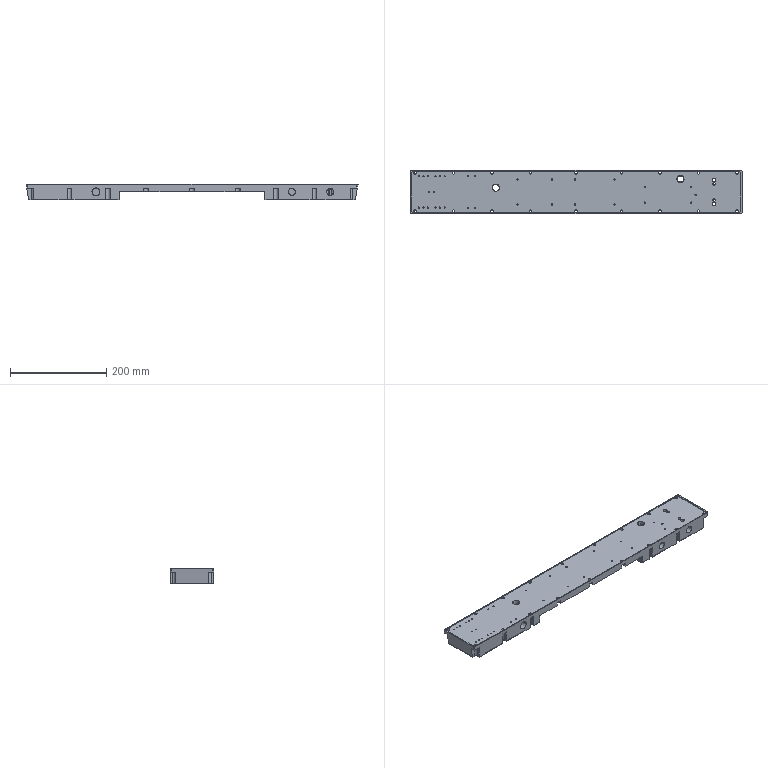CAM job | Mastercam | mm | 18 operations | part box 691.4 x 90 x 32.6
1. Facing | 24 - 100 平铣刀
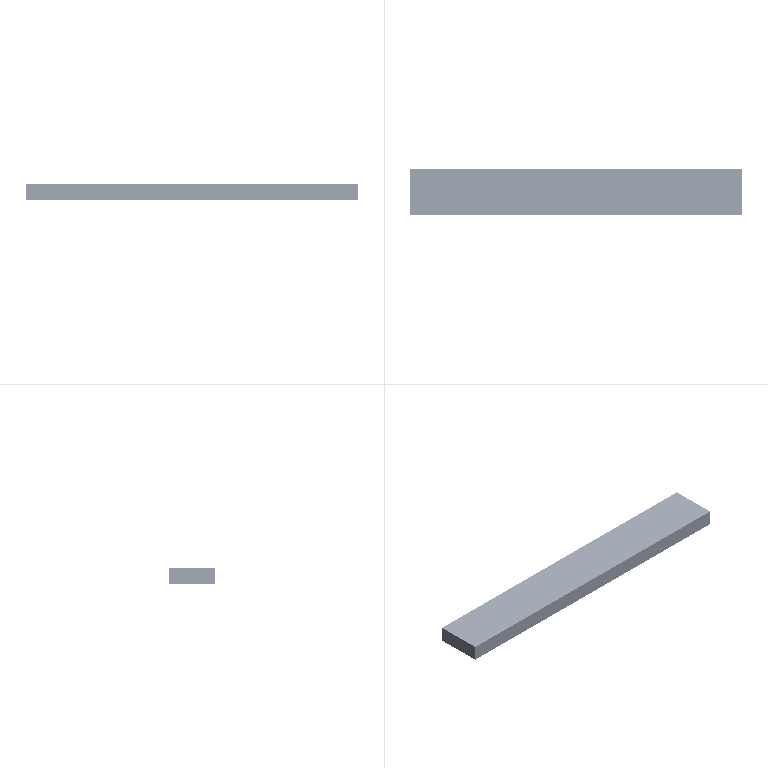2. 2D High Speed (2D Dynamic Mill) | 13 - 16 平铣刀
3. 2D High Speed (2D Area Mill) | 13 - 16 平铣刀
4. Contour (Remachining) | 8 - 8 平铣刀
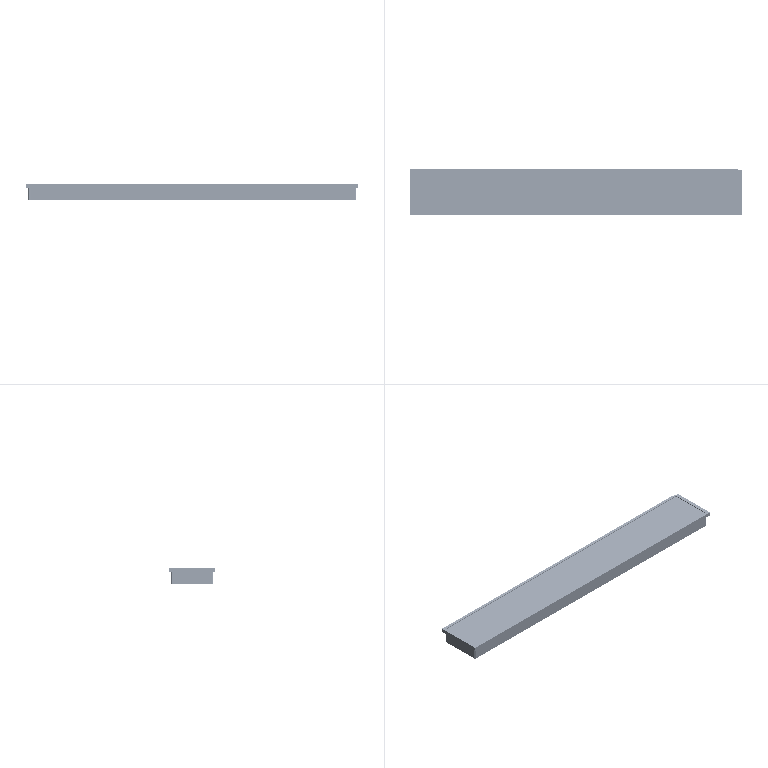5. 2D High Speed (2D Area Mill) | 8 - 8 平铣刀
6. Contour (2D) | 8 - 8 平铣刀
7. Contour (2D) | 16 - 16 平铣刀
8. Drill/Counterbore | 5 - 4 倒角刀
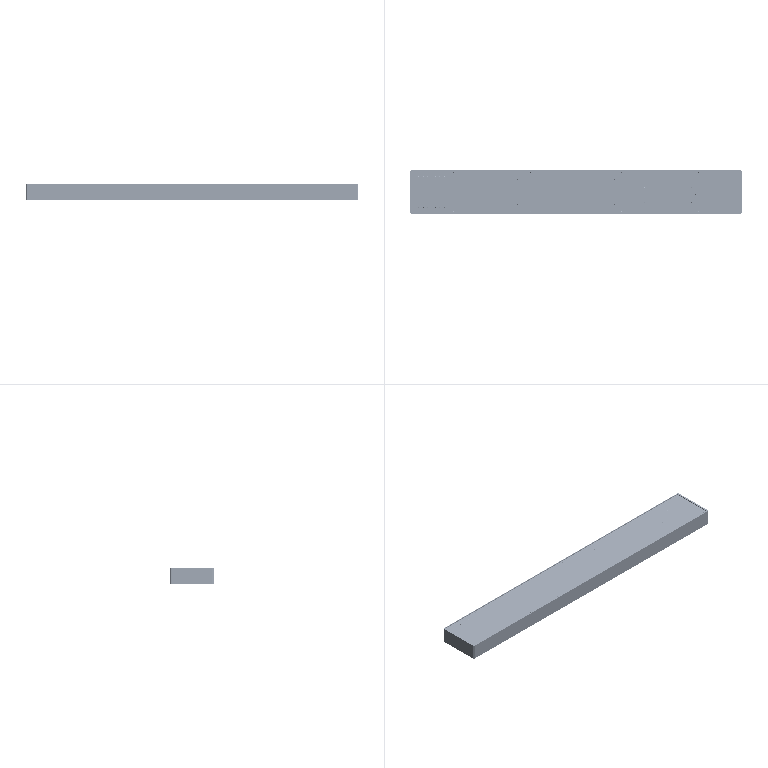9. Peck Drill | 1 - 8 钻头
10. Contour (2D chamfer) | 5 - 4 倒角刀
11. Facing | 24 - 100 平铣刀
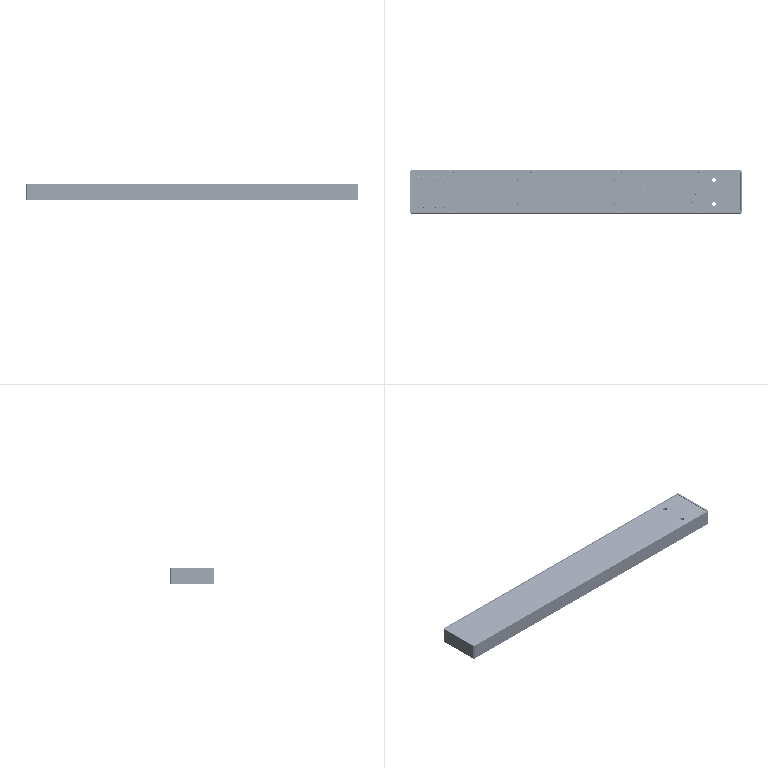12. 2D High Speed (2D Area Mill) | 13 - 16 平铣刀
13. Contour (Ramp) | 9 - 10 平铣刀
14. Contour (Ramp) | 10 - 10 平铣刀
15. Contour (Ramp) | 8 - 8 平铣刀
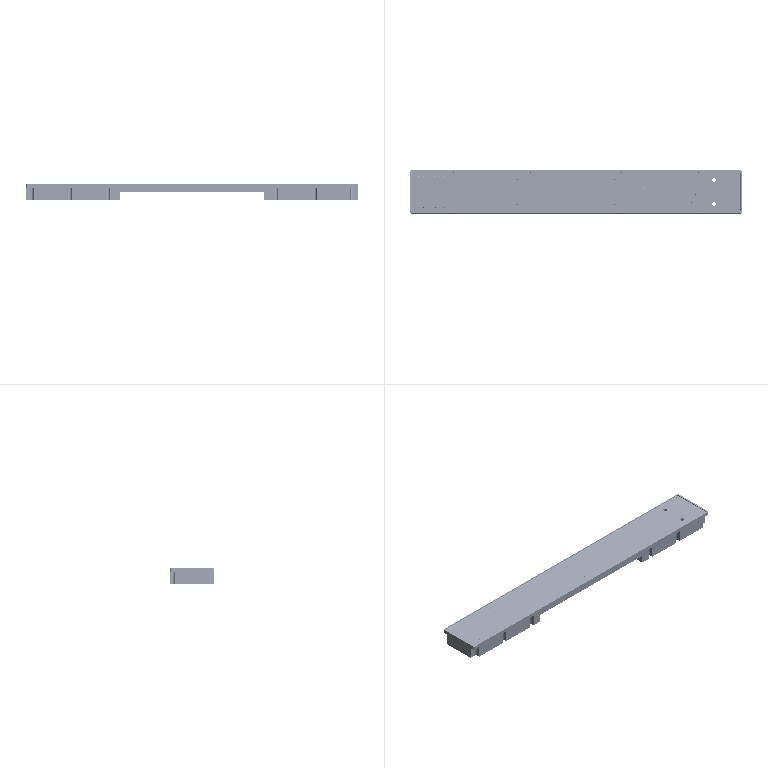16. Contour (2D) | 8 - 8 平铣刀
17. Contour (Ramp) | 8 - 8 平铣刀
18. Contour (2D) | 8 - 8 平铣刀